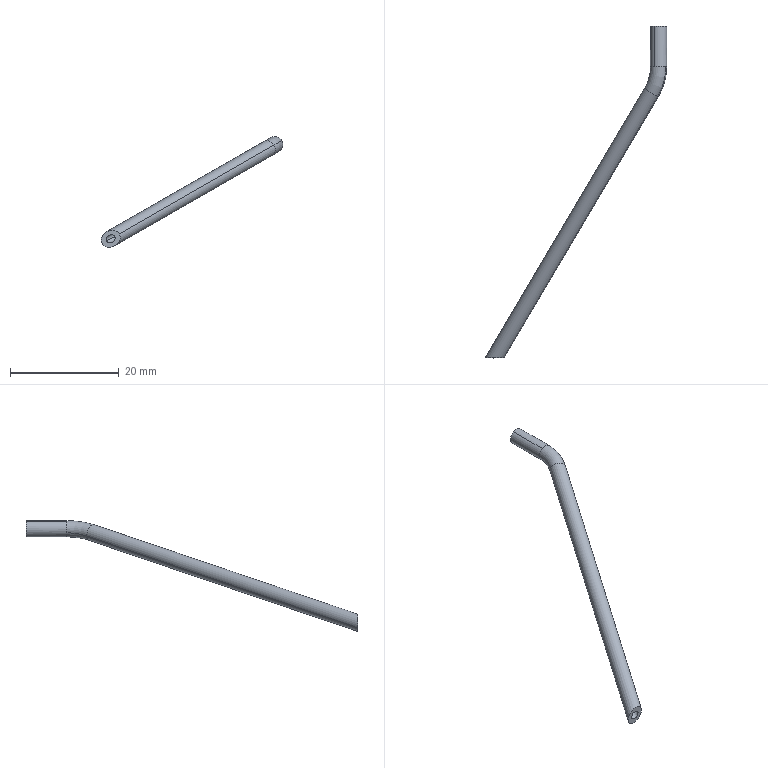Component | SolidWorks | WireFeedingHose-1 | 1 solid | 14 faces | box 33.45 x 61.16 x 20.41 mm | volume 397 mm3 | cylinder 8 | torus 4 | plane 2 | commonest cylinder face diameters 1.4 x4 3 x4
STEP:
#1=CARTESIAN_POINT('',(1.454,-0.3738,7.306));
#2=VERTEX_POINT('',#1);
#3=CARTESIAN_POINT('',(1.491,-0.3738,7.296));
#4=VERTEX_POINT('',#3);
#5=CARTESIAN_POINT('',(1.467,-0.3738,7.282));
#6=DIRECTION('',(-0.,1.,0.));
#7=DIRECTION('',(0.4976,0.,-0.8674));
#8=AXIS2_PLACEMENT_3D('',#5,#6,#7);
#9=CIRCLE('',#8,0.02756);
#10=EDGE_CURVE('',#2,#4,#9,.T.);
#11=ORIENTED_EDGE('',*,*,#10,.T.);
#12=CARTESIAN_POINT('',(1.44,-0.5665,7.267));
#13=VERTEX_POINT('',#12);
#14=CARTESIAN_POINT('',(1.194,-0.3738,7.126));
#15=DIRECTION('',(0.4976,0.,-0.8674));
#16=DIRECTION('',(-0.8674,0.,-0.4976));
#17=AXIS2_PLACEMENT_3D('',#14,#15,#16);
#18=CIRCLE('',#17,0.3425);
#19=EDGE_CURVE('',#4,#13,#18,.T.);
#20=ORIENTED_EDGE('',*,*,#19,.T.);
#21=CARTESIAN_POINT('',(1.4,-0.5355,7.244));
#22=VERTEX_POINT('',#21);
#23=CARTESIAN_POINT('',(1.42,-0.551,7.255));
#24=DIRECTION('',(0.4881,0.8266,0.28));
#25=DIRECTION('',(-0.717,0.5627,-0.4113));
#26=AXIS2_PLACEMENT_3D('',#23,#24,#25);
#27=CIRCLE('',#26,0.02756);
#28=EDGE_CURVE('',#22,#13,#27,.T.);
#29=ORIENTED_EDGE('',*,*,#28,.F.);
#30=CARTESIAN_POINT('',(1.443,-0.3738,7.269));
#31=VERTEX_POINT('',#30);
#32=CARTESIAN_POINT('',(1.194,-0.3738,7.126));
#33=DIRECTION('',(0.4976,0.,-0.8674));
#34=DIRECTION('',(-0.8674,0.,-0.4976));
#35=AXIS2_PLACEMENT_3D('',#32,#33,#34);
#36=CIRCLE('',#35,0.2874);
#37=EDGE_CURVE('',#31,#22,#36,.T.);
#38=ORIENTED_EDGE('',*,*,#37,.F.);
#39=CARTESIAN_POINT('',(1.467,-0.3738,7.282));
#40=DIRECTION('',(-0.,1.,0.));
#41=DIRECTION('',(0.4976,0.,-0.8674));
#42=AXIS2_PLACEMENT_3D('',#39,#40,#41);
#43=CIRCLE('',#42,0.02756);
#44=EDGE_CURVE('',#31,#2,#43,.T.);
#45=ORIENTED_EDGE('',*,*,#44,.T.);
#46=EDGE_LOOP('',(#11,#20,#29,#38,#45));
#47=FACE_OUTER_BOUND('',#46,.T.);
#48=CARTESIAN_POINT('',(1.194,-0.3738,7.126));
#49=DIRECTION('',(0.4976,0.,-0.8674));
#50=DIRECTION('',(-0.8674,0.,-0.4976));
#51=AXIS2_PLACEMENT_3D('',#48,#49,#50);
#52=TOROIDAL_SURFACE('',#51,0.315,0.02756);
#53=ADVANCED_FACE('',(#47),#52,.F.);
#54=CARTESIAN_POINT('',(1.519,-0.3738,7.312));
#55=VERTEX_POINT('',#54);
#56=CARTESIAN_POINT('',(1.497,-0.3738,7.231));
#57=VERTEX_POINT('',#56);
#58=CARTESIAN_POINT('',(1.467,-0.3738,7.282));
#59=DIRECTION('',(0.,1.,0.));
#60=DIRECTION('',(-0.8674,0.,-0.4976));
#61=AXIS2_PLACEMENT_3D('',#58,#59,#60);
#62=CIRCLE('',#61,0.05906);
#63=EDGE_CURVE('',#55,#57,#62,.T.);
#64=ORIENTED_EDGE('',*,*,#63,.F.);
#65=CARTESIAN_POINT('',(1.462,-0.5842,7.279));
#66=VERTEX_POINT('',#65);
#67=CARTESIAN_POINT('',(1.194,-0.3738,7.126));
#68=DIRECTION('',(0.4976,0.,-0.8674));
#69=DIRECTION('',(-0.8674,0.,-0.4976));
#70=AXIS2_PLACEMENT_3D('',#67,#68,#69);
#71=CIRCLE('',#70,0.374);
#72=EDGE_CURVE('',#55,#66,#71,.T.);
#73=ORIENTED_EDGE('',*,*,#72,.T.);
#74=CARTESIAN_POINT('',(1.378,-0.5178,7.231));
#75=VERTEX_POINT('',#74);
#76=CARTESIAN_POINT('',(1.42,-0.551,7.255));
#77=DIRECTION('',(0.4881,0.8266,0.28));
#78=DIRECTION('',(-0.717,0.5627,-0.4113));
#79=AXIS2_PLACEMENT_3D('',#76,#77,#78);
#80=CIRCLE('',#79,0.05906);
#81=EDGE_CURVE('',#66,#75,#80,.T.);
#82=ORIENTED_EDGE('',*,*,#81,.T.);
#83=CARTESIAN_POINT('',(1.416,-0.3738,7.253));
#84=VERTEX_POINT('',#83);
#85=CARTESIAN_POINT('',(1.194,-0.3738,7.126));
#86=DIRECTION('',(0.4976,0.,-0.8674));
#87=DIRECTION('',(-0.8674,0.,-0.4976));
#88=AXIS2_PLACEMENT_3D('',#85,#86,#87);
#89=CIRCLE('',#88,0.2559);
#90=EDGE_CURVE('',#84,#75,#89,.T.);
#91=ORIENTED_EDGE('',*,*,#90,.F.);
#92=CARTESIAN_POINT('',(1.467,-0.3738,7.282));
#93=DIRECTION('',(0.,1.,0.));
#94=DIRECTION('',(-0.8674,0.,-0.4976));
#95=AXIS2_PLACEMENT_3D('',#92,#93,#94);
#96=CIRCLE('',#95,0.05906);
#97=EDGE_CURVE('',#57,#84,#96,.T.);
#98=ORIENTED_EDGE('',*,*,#97,.F.);
#99=EDGE_LOOP('',(#64,#73,#82,#91,#98));
#100=FACE_OUTER_BOUND('',#99,.T.);
#101=CARTESIAN_POINT('',(1.194,-0.3738,7.126));
#102=DIRECTION('',(0.4976,0.,-0.8674));
#103=DIRECTION('',(-0.8674,-0.,-0.4976));
#104=AXIS2_PLACEMENT_3D('',#101,#102,#103);
#105=TOROIDAL_SURFACE('',#104,0.315,0.05906);
#106=ADVANCED_FACE('',(#100),#105,.T.);
#107=CARTESIAN_POINT('',(1.42,-0.551,7.255));
#108=DIRECTION('',(0.4881,0.8266,0.28));
#109=DIRECTION('',(-0.717,0.5627,-0.4113));
#110=AXIS2_PLACEMENT_3D('',#107,#108,#109);
#111=CIRCLE('',#110,0.02756);
#112=EDGE_CURVE('',#13,#22,#111,.T.);
#113=ORIENTED_EDGE('',*,*,#112,.T.);
#114=CARTESIAN_POINT('',(0.2491,-2.485,6.584));
#115=VERTEX_POINT('',#114);
#116=CARTESIAN_POINT('',(1.4,-0.5355,7.244));
#117=DIRECTION('',(-0.4881,-0.8266,-0.28));
#118=VECTOR('',#117,39.37);
#119=LINE('',#116,#118);
#120=EDGE_CURVE('',#22,#115,#119,.T.);
#121=ORIENTED_EDGE('',*,*,#120,.T.);
#122=CARTESIAN_POINT('',(0.307,-2.485,6.617));
#123=VERTEX_POINT('',#122);
#124=CARTESIAN_POINT('',(0.307,-2.485,6.617));
#125=CARTESIAN_POINT('',(0.3344,-2.485,6.569));
#126=CARTESIAN_POINT('',(0.2766,-2.485,6.536));
#127=CARTESIAN_POINT('',(0.2491,-2.485,6.584));
#128=(BOUNDED_CURVE()B_SPLINE_CURVE(3,(#124,#125,#126,#127),.UNSPECIFIED.,.F.,.T.)B_SPLINE_CURVE_WITH_KNOTS((4,4),(3.142,6.283),.UNSPECIFIED.)CURVE()GEOMETRIC_REPRESENTATION_ITEM()RATIONAL_B_SPLINE_CURVE((1.,0.3333,0.3333,1.))REPRESENTATION_ITEM(''));
#129=EDGE_CURVE('',#123,#115,#128,.T.);
#130=ORIENTED_EDGE('',*,*,#129,.F.);
#131=CARTESIAN_POINT('',(1.44,-0.5665,7.267));
#132=DIRECTION('',(-0.4881,-0.8266,-0.28));
#133=VECTOR('',#132,39.37);
#134=LINE('',#131,#133);
#135=EDGE_CURVE('',#13,#123,#134,.T.);
#136=ORIENTED_EDGE('',*,*,#135,.F.);
#137=EDGE_LOOP('',(#113,#121,#130,#136));
#138=FACE_OUTER_BOUND('',#137,.T.);
#139=CARTESIAN_POINT('',(1.42,-0.551,7.255));
#140=DIRECTION('',(-0.4881,-0.8266,-0.28));
#141=DIRECTION('',(0.717,-0.5627,0.4113));
#142=AXIS2_PLACEMENT_3D('',#139,#140,#141);
#143=CYLINDRICAL_SURFACE('',#142,0.02756);
#144=ADVANCED_FACE('',(#138),#143,.F.);
#145=CARTESIAN_POINT('',(1.481,-0.0771,7.258));
#146=VERTEX_POINT('',#145);
#147=CARTESIAN_POINT('',(1.454,-0.0771,7.306));
#148=VERTEX_POINT('',#147);
#149=CARTESIAN_POINT('',(1.467,-0.0771,7.282));
#150=DIRECTION('',(0.,1.,0.));
#151=DIRECTION('',(-0.8674,0.,-0.4976));
#152=AXIS2_PLACEMENT_3D('',#149,#150,#151);
#153=CIRCLE('',#152,0.02756);
#154=EDGE_CURVE('',#146,#148,#153,.T.);
#155=ORIENTED_EDGE('',*,*,#154,.T.);
#156=CARTESIAN_POINT('',(1.454,-0.0771,7.306));
#157=DIRECTION('',(0.,-1.,-0.));
#158=VECTOR('',#157,39.37);
#159=LINE('',#156,#158);
#160=EDGE_CURVE('',#148,#2,#159,.T.);
#161=ORIENTED_EDGE('',*,*,#160,.T.);
#162=ORIENTED_EDGE('',*,*,#44,.F.);
#163=CARTESIAN_POINT('',(1.481,-0.3738,7.258));
#164=VERTEX_POINT('',#163);
#165=CARTESIAN_POINT('',(1.467,-0.3738,7.282));
#166=DIRECTION('',(-0.,1.,0.));
#167=DIRECTION('',(0.4976,0.,-0.8674));
#168=AXIS2_PLACEMENT_3D('',#165,#166,#167);
#169=CIRCLE('',#168,0.02756);
#170=EDGE_CURVE('',#164,#31,#169,.T.);
#171=ORIENTED_EDGE('',*,*,#170,.F.);
#172=CARTESIAN_POINT('',(1.481,-0.0771,7.258));
#173=DIRECTION('',(0.,-1.,-0.));
#174=VECTOR('',#173,39.37);
#175=LINE('',#172,#174);
#176=EDGE_CURVE('',#146,#164,#175,.T.);
#177=ORIENTED_EDGE('',*,*,#176,.F.);
#178=EDGE_LOOP('',(#155,#161,#162,#171,#177));
#179=FACE_OUTER_BOUND('',#178,.T.);
#180=CARTESIAN_POINT('',(1.467,-0.0771,7.282));
#181=DIRECTION('',(0.,-1.,-0.));
#182=DIRECTION('',(0.4976,0.,-0.8674));
#183=AXIS2_PLACEMENT_3D('',#180,#181,#182);
#184=CYLINDRICAL_SURFACE('',#183,0.02756);
#185=ADVANCED_FACE('',(#179),#184,.F.);
#186=CARTESIAN_POINT('',(1.42,-0.551,7.255));
#187=DIRECTION('',(0.4881,0.8266,0.28));
#188=DIRECTION('',(-0.717,0.5627,-0.4113));
#189=AXIS2_PLACEMENT_3D('',#186,#187,#188);
#190=CIRCLE('',#189,0.05906);
#191=EDGE_CURVE('',#75,#66,#190,.T.);
#192=ORIENTED_EDGE('',*,*,#191,.F.);
#193=CARTESIAN_POINT('',(0.2161,-2.485,6.565));
#194=VERTEX_POINT('',#193);
#195=CARTESIAN_POINT('',(1.378,-0.5178,7.231));
#196=DIRECTION('',(-0.4881,-0.8266,-0.28));
#197=VECTOR('',#196,39.37);
#198=LINE('',#195,#197);
#199=EDGE_CURVE('',#75,#194,#198,.T.);
#200=ORIENTED_EDGE('',*,*,#199,.T.);
#201=CARTESIAN_POINT('',(0.34,-2.485,6.636));
#202=VERTEX_POINT('',#201);
#203=CARTESIAN_POINT('',(0.2161,-2.485,6.565));
#204=CARTESIAN_POINT('',(0.1573,-2.485,6.667));
#205=CARTESIAN_POINT('',(0.2813,-2.485,6.738));
#206=CARTESIAN_POINT('',(0.34,-2.485,6.636));
#207=(BOUNDED_CURVE()B_SPLINE_CURVE(3,(#203,#204,#205,#206),.UNSPECIFIED.,.F.,.F.)B_SPLINE_CURVE_WITH_KNOTS((4,4),(0.,3.142),.UNSPECIFIED.)CURVE()GEOMETRIC_REPRESENTATION_ITEM()RATIONAL_B_SPLINE_CURVE((1.,0.3333,0.3333,1.))REPRESENTATION_ITEM(''));
#208=EDGE_CURVE('',#194,#202,#207,.T.);
#209=ORIENTED_EDGE('',*,*,#208,.T.);
#210=CARTESIAN_POINT('',(1.462,-0.5842,7.279));
#211=DIRECTION('',(-0.4881,-0.8266,-0.28));
#212=VECTOR('',#211,39.37);
#213=LINE('',#210,#212);
#214=EDGE_CURVE('',#66,#202,#213,.T.);
#215=ORIENTED_EDGE('',*,*,#214,.F.);
#216=EDGE_LOOP('',(#192,#200,#209,#215));
#217=FACE_OUTER_BOUND('',#216,.T.);
#218=CARTESIAN_POINT('',(1.42,-0.551,7.255));
#219=DIRECTION('',(-0.4881,-0.8266,-0.28));
#220=DIRECTION('',(0.717,-0.5627,0.4113));
#221=AXIS2_PLACEMENT_3D('',#218,#219,#220);
#222=CYLINDRICAL_SURFACE('',#221,0.05906);
#223=ADVANCED_FACE('',(#217),#222,.T.);
#224=CARTESIAN_POINT('',(1.438,-0.0771,7.334));
#225=VERTEX_POINT('',#224);
#226=CARTESIAN_POINT('',(1.497,-0.0771,7.231));
#227=VERTEX_POINT('',#226);
#228=CARTESIAN_POINT('',(1.467,-0.0771,7.282));
#229=DIRECTION('',(0.,1.,0.));
#230=DIRECTION('',(-0.8674,0.,-0.4976));
#231=AXIS2_PLACEMENT_3D('',#228,#229,#230);
#232=CIRCLE('',#231,0.05906);
#233=EDGE_CURVE('',#225,#227,#232,.T.);
#234=ORIENTED_EDGE('',*,*,#233,.F.);
#235=CARTESIAN_POINT('',(1.438,-0.3738,7.334));
#236=VERTEX_POINT('',#235);
#237=CARTESIAN_POINT('',(1.438,-0.0771,7.334));
#238=DIRECTION('',(0.,-1.,-0.));
#239=VECTOR('',#238,39.37);
#240=LINE('',#237,#239);
#241=EDGE_CURVE('',#225,#236,#240,.T.);
#242=ORIENTED_EDGE('',*,*,#241,.T.);
#243=CARTESIAN_POINT('',(1.467,-0.3738,7.282));
#244=DIRECTION('',(0.,1.,0.));
#245=DIRECTION('',(-0.8674,0.,-0.4976));
#246=AXIS2_PLACEMENT_3D('',#243,#244,#245);
#247=CIRCLE('',#246,0.05906);
#248=EDGE_CURVE('',#236,#55,#247,.T.);
#249=ORIENTED_EDGE('',*,*,#248,.T.);
#250=ORIENTED_EDGE('',*,*,#63,.T.);
#251=CARTESIAN_POINT('',(1.497,-0.0771,7.231));
#252=DIRECTION('',(0.,-1.,-0.));
#253=VECTOR('',#252,39.37);
#254=LINE('',#251,#253);
#255=EDGE_CURVE('',#227,#57,#254,.T.);
#256=ORIENTED_EDGE('',*,*,#255,.F.);
#257=EDGE_LOOP('',(#234,#242,#249,#250,#256));
#258=FACE_OUTER_BOUND('',#257,.T.);
#259=CARTESIAN_POINT('',(1.467,-0.0771,7.282));
#260=DIRECTION('',(0.,-1.,-0.));
#261=DIRECTION('',(0.4976,0.,-0.8674));
#262=AXIS2_PLACEMENT_3D('',#259,#260,#261);
#263=CYLINDRICAL_SURFACE('',#262,0.05906);
#264=ADVANCED_FACE('',(#258),#263,.T.);
#265=ORIENTED_EDGE('',*,*,#199,.F.);
#266=ORIENTED_EDGE('',*,*,#81,.F.);
#267=ORIENTED_EDGE('',*,*,#214,.T.);
#268=CARTESIAN_POINT('',(0.34,-2.485,6.636));
#269=CARTESIAN_POINT('',(0.3988,-2.485,6.533));
#270=CARTESIAN_POINT('',(0.2749,-2.485,6.462));
#271=CARTESIAN_POINT('',(0.2161,-2.485,6.565));
#272=(BOUNDED_CURVE()B_SPLINE_CURVE(3,(#268,#269,#270,#271),.UNSPECIFIED.,.F.,.F.)B_SPLINE_CURVE_WITH_KNOTS((4,4),(3.142,6.283),.UNSPECIFIED.)CURVE()GEOMETRIC_REPRESENTATION_ITEM()RATIONAL_B_SPLINE_CURVE((1.,0.3333,0.3333,1.))REPRESENTATION_ITEM(''));
#273=EDGE_CURVE('',#202,#194,#272,.T.);
#274=ORIENTED_EDGE('',*,*,#273,.T.);
#275=EDGE_LOOP('',(#265,#266,#267,#274));
#276=FACE_OUTER_BOUND('',#275,.T.);
#277=CARTESIAN_POINT('',(1.42,-0.551,7.255));
#278=DIRECTION('',(-0.4881,-0.8266,-0.28));
#279=DIRECTION('',(0.717,-0.5627,0.4113));
#280=AXIS2_PLACEMENT_3D('',#277,#278,#279);
#281=CYLINDRICAL_SURFACE('',#280,0.05906);
#282=ADVANCED_FACE('',(#276),#281,.T.);
#283=ORIENTED_EDGE('',*,*,#72,.F.);
#284=ORIENTED_EDGE('',*,*,#248,.F.);
#285=CARTESIAN_POINT('',(1.467,-0.3738,7.282));
#286=DIRECTION('',(0.,1.,0.));
#287=DIRECTION('',(-0.8674,0.,-0.4976));
#288=AXIS2_PLACEMENT_3D('',#285,#286,#287);
#289=CIRCLE('',#288,0.05906);
#290=EDGE_CURVE('',#84,#236,#289,.T.);
#291=ORIENTED_EDGE('',*,*,#290,.F.);
#292=ORIENTED_EDGE('',*,*,#90,.T.);
#293=ORIENTED_EDGE('',*,*,#191,.T.);
#294=EDGE_LOOP('',(#283,#284,#291,#292,#293));
#295=FACE_OUTER_BOUND('',#294,.T.);
#296=CARTESIAN_POINT('',(1.194,-0.3738,7.126));
#297=DIRECTION('',(0.4976,0.,-0.8674));
#298=DIRECTION('',(-0.8674,-0.,-0.4976));
#299=AXIS2_PLACEMENT_3D('',#296,#297,#298);
#300=TOROIDAL_SURFACE('',#299,0.315,0.05906);
#301=ADVANCED_FACE('',(#295),#300,.T.);
#302=ORIENTED_EDGE('',*,*,#241,.F.);
#303=CARTESIAN_POINT('',(1.467,-0.0771,7.282));
#304=DIRECTION('',(0.,1.,0.));
#305=DIRECTION('',(-0.8674,0.,-0.4976));
#306=AXIS2_PLACEMENT_3D('',#303,#304,#305);
#307=CIRCLE('',#306,0.05906);
#308=EDGE_CURVE('',#227,#225,#307,.T.);
#309=ORIENTED_EDGE('',*,*,#308,.F.);
#310=ORIENTED_EDGE('',*,*,#255,.T.);
#311=ORIENTED_EDGE('',*,*,#97,.T.);
#312=ORIENTED_EDGE('',*,*,#290,.T.);
#313=EDGE_LOOP('',(#302,#309,#310,#311,#312));
#314=FACE_OUTER_BOUND('',#313,.T.);
#315=CARTESIAN_POINT('',(1.467,-0.0771,7.282));
#316=DIRECTION('',(0.,-1.,-0.));
#317=DIRECTION('',(0.4976,0.,-0.8674));
#318=AXIS2_PLACEMENT_3D('',#315,#316,#317);
#319=CYLINDRICAL_SURFACE('',#318,0.05906);
#320=ADVANCED_FACE('',(#314),#319,.T.);
#321=ORIENTED_EDGE('',*,*,#154,.F.);
#322=CARTESIAN_POINT('',(1.467,-0.0771,7.282));
#323=DIRECTION('',(0.,1.,0.));
#324=DIRECTION('',(-0.8674,0.,-0.4976));
#325=AXIS2_PLACEMENT_3D('',#322,#323,#324);
#326=CIRCLE('',#325,0.02756);
#327=EDGE_CURVE('',#148,#146,#326,.T.);
#328=ORIENTED_EDGE('',*,*,#327,.F.);
#329=EDGE_LOOP('',(#321,#328));
#330=FACE_BOUND('',#329,.T.);
#331=ORIENTED_EDGE('',*,*,#308,.T.);
#332=ORIENTED_EDGE('',*,*,#233,.T.);
#333=EDGE_LOOP('',(#331,#332));
#334=FACE_OUTER_BOUND('',#333,.T.);
#335=CARTESIAN_POINT('',(1.467,-0.0771,7.282));
#336=DIRECTION('',(-0.,1.,0.));
#337=DIRECTION('',(-0.8674,0.,-0.4976));
#338=AXIS2_PLACEMENT_3D('',#335,#336,#337);
#339=PLANE('',#338);
#340=ADVANCED_FACE('',(#330,#334),#339,.T.);
#341=ORIENTED_EDGE('',*,*,#120,.F.);
#342=ORIENTED_EDGE('',*,*,#28,.T.);
#343=ORIENTED_EDGE('',*,*,#135,.T.);
#344=CARTESIAN_POINT('',(0.2491,-2.485,6.584));
#345=CARTESIAN_POINT('',(0.2217,-2.485,6.631));
#346=CARTESIAN_POINT('',(0.2796,-2.485,6.665));
#347=CARTESIAN_POINT('',(0.307,-2.485,6.617));
#348=(BOUNDED_CURVE()B_SPLINE_CURVE(3,(#344,#345,#346,#347),.UNSPECIFIED.,.F.,.F.)B_SPLINE_CURVE_WITH_KNOTS((4,4),(0.,3.142),.UNSPECIFIED.)CURVE()GEOMETRIC_REPRESENTATION_ITEM()RATIONAL_B_SPLINE_CURVE((1.,0.3333,0.3333,1.))REPRESENTATION_ITEM(''));
#349=EDGE_CURVE('',#115,#123,#348,.T.);
#350=ORIENTED_EDGE('',*,*,#349,.F.);
#351=EDGE_LOOP('',(#341,#342,#343,#350));
#352=FACE_OUTER_BOUND('',#351,.T.);
#353=CARTESIAN_POINT('',(1.42,-0.551,7.255));
#354=DIRECTION('',(-0.4881,-0.8266,-0.28));
#355=DIRECTION('',(0.717,-0.5627,0.4113));
#356=AXIS2_PLACEMENT_3D('',#353,#354,#355);
#357=CYLINDRICAL_SURFACE('',#356,0.02756);
#358=ADVANCED_FACE('',(#352),#357,.F.);
#359=ORIENTED_EDGE('',*,*,#19,.F.);
#360=CARTESIAN_POINT('',(1.467,-0.3738,7.282));
#361=DIRECTION('',(-0.,1.,0.));
#362=DIRECTION('',(0.4976,0.,-0.8674));
#363=AXIS2_PLACEMENT_3D('',#360,#361,#362);
#364=CIRCLE('',#363,0.02756);
#365=EDGE_CURVE('',#4,#164,#364,.T.);
#366=ORIENTED_EDGE('',*,*,#365,.T.);
#367=ORIENTED_EDGE('',*,*,#170,.T.);
#368=ORIENTED_EDGE('',*,*,#37,.T.);
#369=ORIENTED_EDGE('',*,*,#112,.F.);
#370=EDGE_LOOP('',(#359,#366,#367,#368,#369));
#371=FACE_OUTER_BOUND('',#370,.T.);
#372=CARTESIAN_POINT('',(1.194,-0.3738,7.126));
#373=DIRECTION('',(0.4976,0.,-0.8674));
#374=DIRECTION('',(-0.8674,0.,-0.4976));
#375=AXIS2_PLACEMENT_3D('',#372,#373,#374);
#376=TOROIDAL_SURFACE('',#375,0.315,0.02756);
#377=ADVANCED_FACE('',(#371),#376,.F.);
#378=ORIENTED_EDGE('',*,*,#160,.F.);
#379=ORIENTED_EDGE('',*,*,#327,.T.);
#380=ORIENTED_EDGE('',*,*,#176,.T.);
#381=ORIENTED_EDGE('',*,*,#365,.F.);
#382=ORIENTED_EDGE('',*,*,#10,.F.);
#383=EDGE_LOOP('',(#378,#379,#380,#381,#382));
#384=FACE_OUTER_BOUND('',#383,.T.);
#385=CARTESIAN_POINT('',(1.467,-0.0771,7.282));
#386=DIRECTION('',(0.,-1.,-0.));
#387=DIRECTION('',(0.4976,0.,-0.8674));
#388=AXIS2_PLACEMENT_3D('',#385,#386,#387);
#389=CYLINDRICAL_SURFACE('',#388,0.02756);
#390=ADVANCED_FACE('',(#384),#389,.F.);
#391=ORIENTED_EDGE('',*,*,#129,.T.);
#392=ORIENTED_EDGE('',*,*,#349,.T.);
#393=EDGE_LOOP('',(#391,#392));
#394=FACE_BOUND('',#393,.T.);
#395=ORIENTED_EDGE('',*,*,#273,.F.);
#396=ORIENTED_EDGE('',*,*,#208,.F.);
#397=EDGE_LOOP('',(#395,#396));
#398=FACE_OUTER_BOUND('',#397,.T.);
#399=CARTESIAN_POINT('',(0.2455,-2.485,6.513));
#400=DIRECTION('',(-0.,1.,0.));
#401=DIRECTION('',(-0.4976,-0.,0.8674));
#402=AXIS2_PLACEMENT_3D('',#399,#400,#401);
#403=PLANE('',#402);
#404=ADVANCED_FACE('',(#394,#398),#403,.F.);
#405=CLOSED_SHELL('',(#53,#106,#144,#185,#223,#264,#282,#301,#320,#340,#358,#377,#390,#404));
#406=MANIFOLD_SOLID_BREP('',#405);
#407=CARTESIAN_POINT('',(0.,0.,0.));
#408=DIRECTION('',(0.,0.,1.));
#409=DIRECTION('',(1.,0.,0.));
#410=AXIS2_PLACEMENT_3D('',#407,#408,#409);
#411=(LENGTH_UNIT()NAMED_UNIT(*)SI_UNIT($,.METRE.));
#412=LENGTH_MEASURE_WITH_UNIT(LENGTH_MEASURE(0.0254),#411);
#413=DIMENSIONAL_EXPONENTS(1.,0.,0.,0.,0.,0.,0.);
#414=(CONVERSION_BASED_UNIT('',#412)LENGTH_UNIT()NAMED_UNIT(#413));
#415=UNCERTAINTY_MEASURE_WITH_UNIT(LENGTH_MEASURE(0.00001),#414,'','');
#416=(NAMED_UNIT(*)PLANE_ANGLE_UNIT()SI_UNIT($,.RADIAN.));
#417=(NAMED_UNIT(*)SI_UNIT($,.STERADIAN.)SOLID_ANGLE_UNIT());
#418=(GEOMETRIC_REPRESENTATION_CONTEXT(3)GLOBAL_UNCERTAINTY_ASSIGNED_CONTEXT((#415))GLOBAL_UNIT_ASSIGNED_CONTEXT((#414,#416,#417))REPRESENTATION_CONTEXT('',''));
#419=ADVANCED_BREP_SHAPE_REPRESENTATION('',(#406,#410),#418);
#420=COLOUR_RGB('',0.7922,0.8196,0.9333);
#421=FILL_AREA_STYLE_COLOUR('',#420);
#422=FILL_AREA_STYLE('',(#421));
#423=SURFACE_STYLE_FILL_AREA(#422);
#424=SURFACE_SIDE_STYLE('',(#423));
#425=SURFACE_STYLE_USAGE(.BOTH.,#424);
#426=PRESENTATION_STYLE_ASSIGNMENT((#425));
#427=STYLED_ITEM('',(#426),#406);
#428=(LENGTH_UNIT()NAMED_UNIT(*)SI_UNIT($,.METRE.));
#429=LENGTH_MEASURE_WITH_UNIT(LENGTH_MEASURE(0.0254),#428);
#430=DIMENSIONAL_EXPONENTS(1.,0.,0.,0.,0.,0.,0.);
#431=(CONVERSION_BASED_UNIT('',#429)LENGTH_UNIT()NAMED_UNIT(#430));
#432=UNCERTAINTY_MEASURE_WITH_UNIT(LENGTH_MEASURE(0.00001),#431,'','');
#433=(NAMED_UNIT(*)PLANE_ANGLE_UNIT()SI_UNIT($,.RADIAN.));
#434=(NAMED_UNIT(*)SI_UNIT($,.STERADIAN.)SOLID_ANGLE_UNIT());
#435=(GEOMETRIC_REPRESENTATION_CONTEXT(3)GLOBAL_UNCERTAINTY_ASSIGNED_CONTEXT((#432))GLOBAL_UNIT_ASSIGNED_CONTEXT((#431,#433,#434))REPRESENTATION_CONTEXT('',''));
#436=MECHANICAL_DESIGN_GEOMETRIC_PRESENTATION_REPRESENTATION('',(#427),#435);
#437=PRESENTATION_LAYER_ASSIGNMENT('','',(#427));